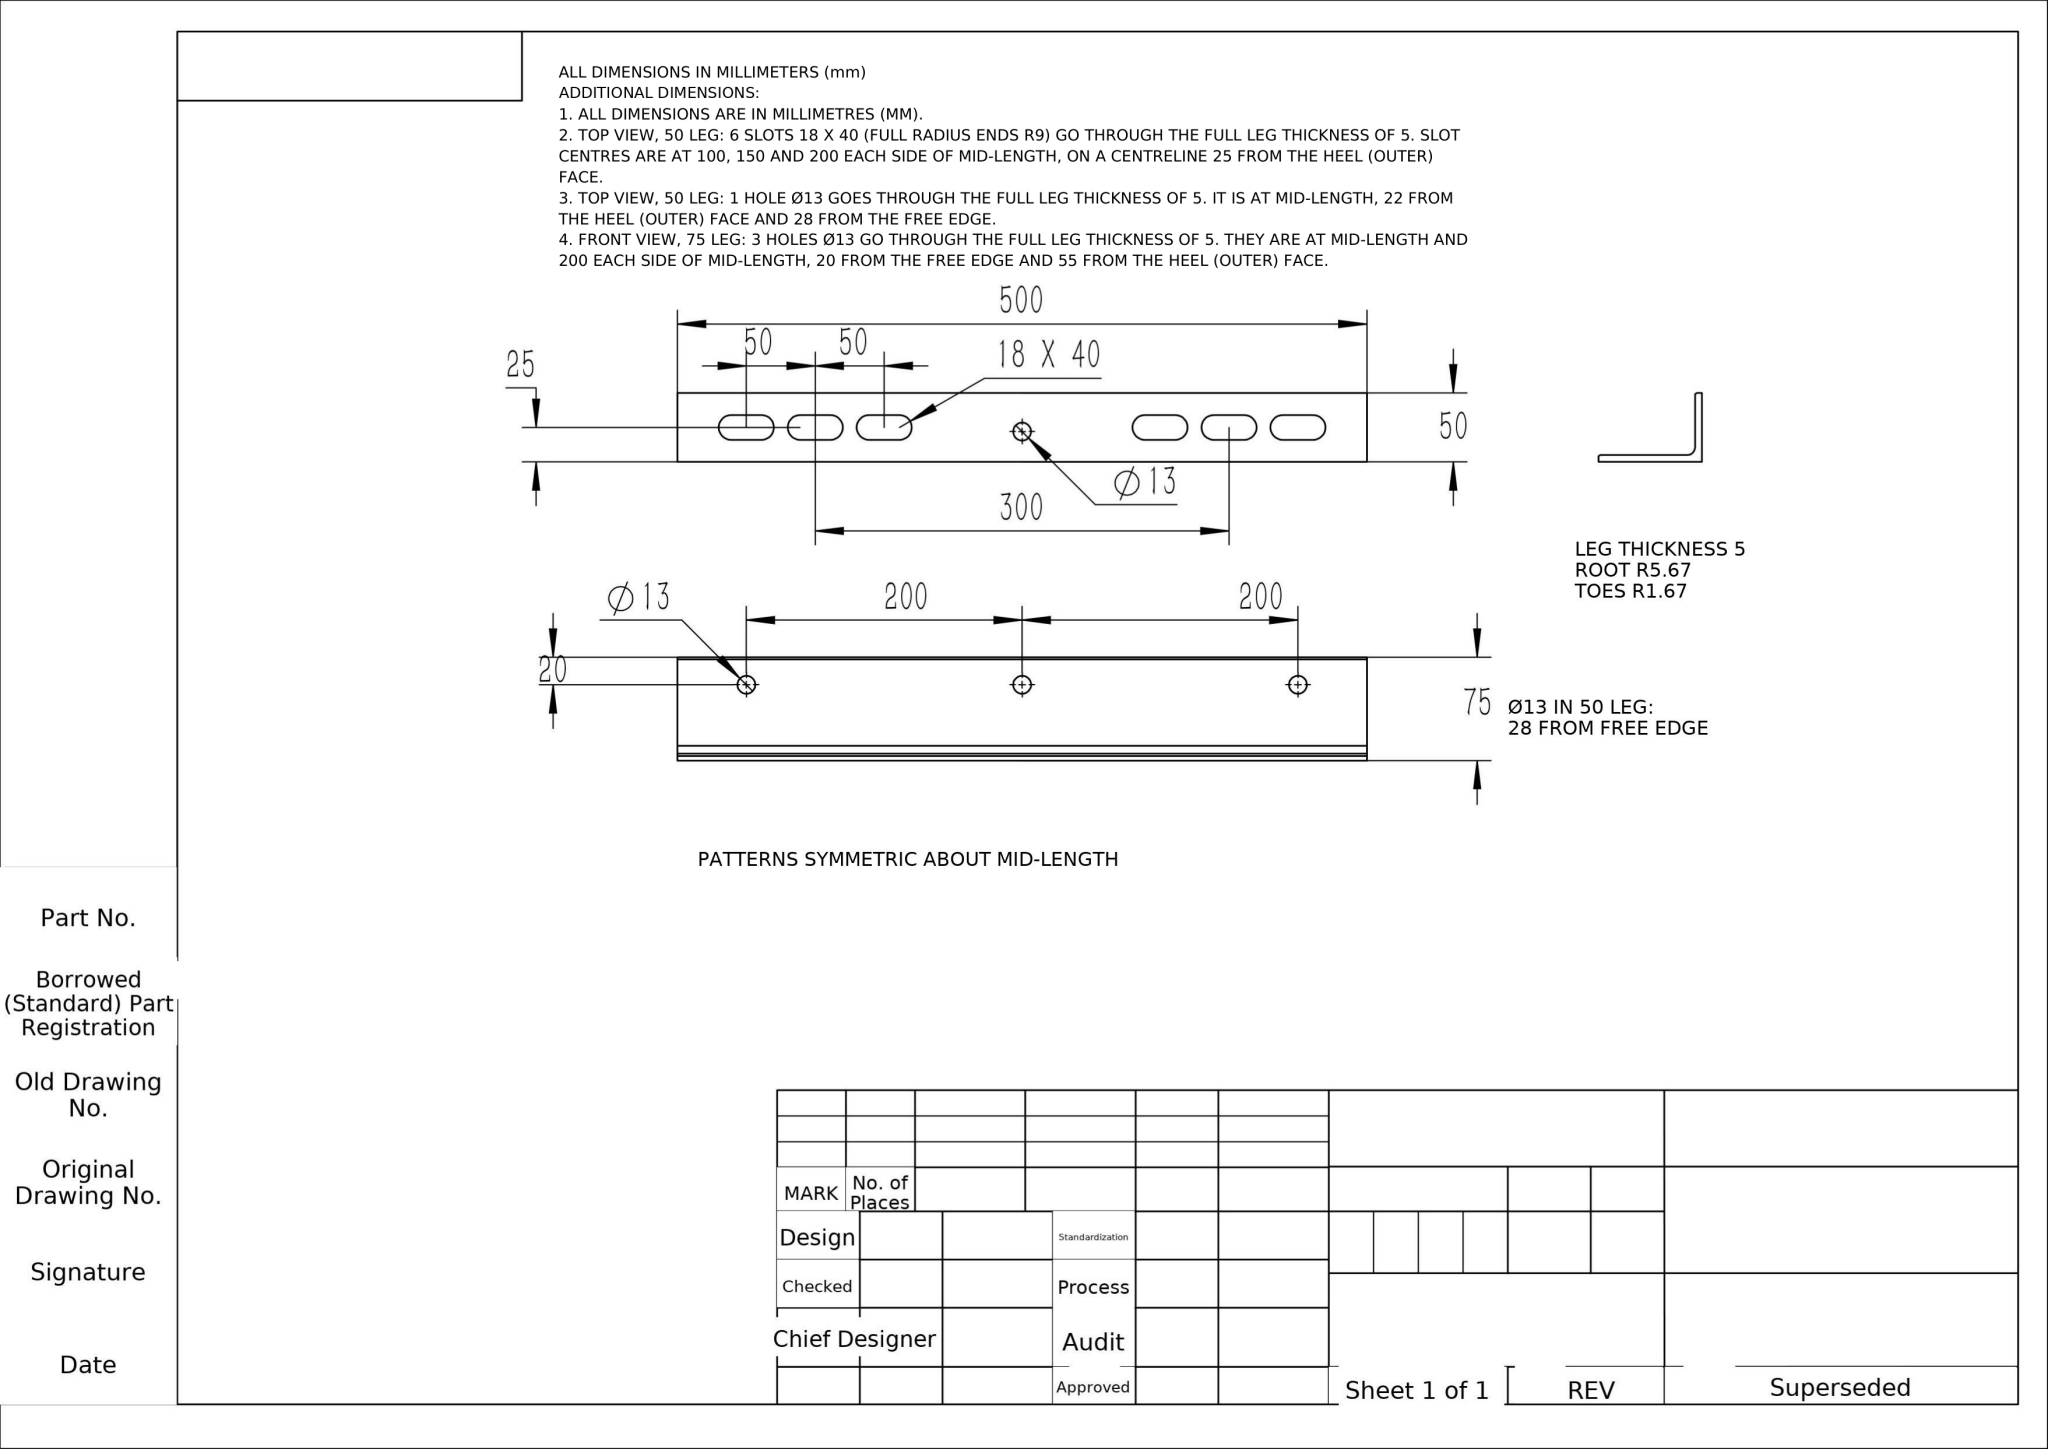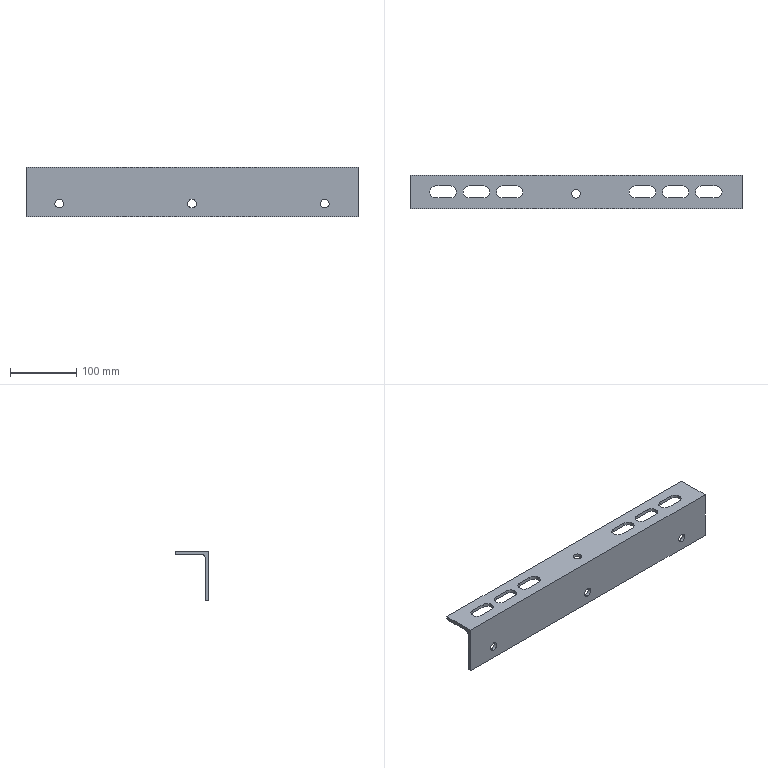Part | NX | mm | Elongated Six-Slot Angle Bracket | 1 solid | 49 faces | box 500 x 50 x 75 mm | volume 280682 mm3 | cylinder 29 | plane 20 | commonest cylinder face diameters 18 x18 13 x8 3.34 x2 11.34 x1